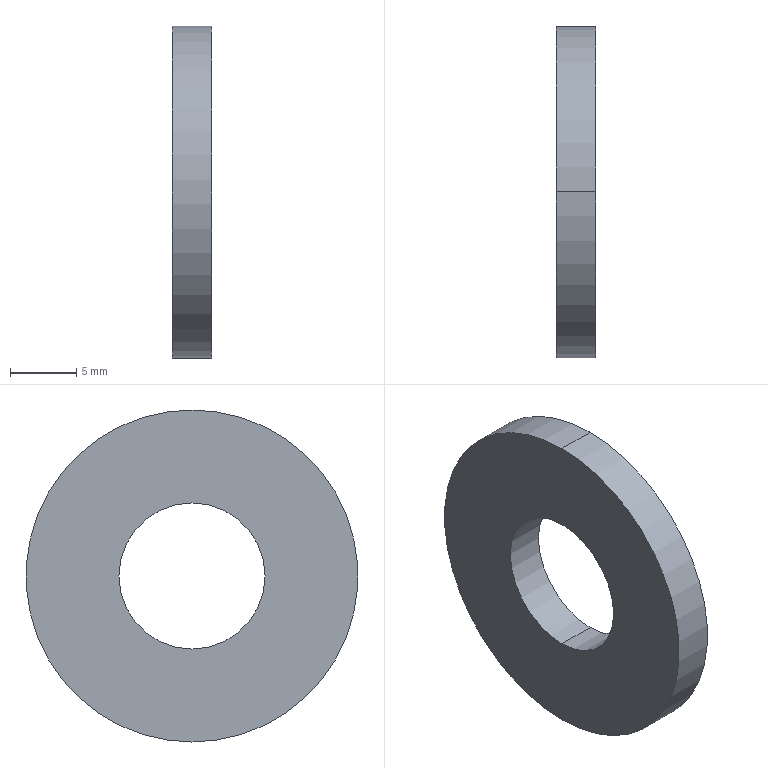Component | SolidWorks | Baffle-1 | 1 solid | 6 faces | box 3 x 25 x 25 mm | volume 1188 mm3 | cylinder 4 | plane 2 | commonest cylinder face diameters 11 x2 25 x2
STEP:
#1=CARTESIAN_POINT('',(7.52,0.7874,3.335));
#2=VERTEX_POINT('',#1);
#3=CARTESIAN_POINT('',(7.52,0.7874,2.902));
#4=VERTEX_POINT('',#3);
#5=CARTESIAN_POINT('',(7.52,0.7874,3.119));
#6=DIRECTION('',(1.,0.,0.));
#7=DIRECTION('',(0.,0.,-1.));
#8=AXIS2_PLACEMENT_3D('',#5,#6,#7);
#9=CIRCLE('',#8,0.2165);
#10=EDGE_CURVE('',#2,#4,#9,.T.);
#11=ORIENTED_EDGE('',*,*,#10,.F.);
#12=CARTESIAN_POINT('',(7.638,0.7874,3.335));
#13=VERTEX_POINT('',#12);
#14=CARTESIAN_POINT('',(7.52,0.7874,3.335));
#15=DIRECTION('',(1.,0.,0.));
#16=VECTOR('',#15,39.37);
#17=LINE('',#14,#16);
#18=EDGE_CURVE('',#2,#13,#17,.T.);
#19=ORIENTED_EDGE('',*,*,#18,.T.);
#20=CARTESIAN_POINT('',(7.638,0.7874,2.902));
#21=VERTEX_POINT('',#20);
#22=CARTESIAN_POINT('',(7.638,0.7874,3.119));
#23=DIRECTION('',(1.,0.,0.));
#24=DIRECTION('',(0.,0.,-1.));
#25=AXIS2_PLACEMENT_3D('',#22,#23,#24);
#26=CIRCLE('',#25,0.2165);
#27=EDGE_CURVE('',#13,#21,#26,.T.);
#28=ORIENTED_EDGE('',*,*,#27,.T.);
#29=CARTESIAN_POINT('',(7.52,0.7874,2.902));
#30=DIRECTION('',(1.,0.,0.));
#31=VECTOR('',#30,39.37);
#32=LINE('',#29,#31);
#33=EDGE_CURVE('',#4,#21,#32,.T.);
#34=ORIENTED_EDGE('',*,*,#33,.F.);
#35=EDGE_LOOP('',(#11,#19,#28,#34));
#36=FACE_OUTER_BOUND('',#35,.T.);
#37=CARTESIAN_POINT('',(7.52,0.7874,3.119));
#38=DIRECTION('',(1.,0.,0.));
#39=DIRECTION('',(0.,0.,-1.));
#40=AXIS2_PLACEMENT_3D('',#37,#38,#39);
#41=CYLINDRICAL_SURFACE('',#40,0.2165);
#42=ADVANCED_FACE('',(#36),#41,.F.);
#43=CARTESIAN_POINT('',(7.52,0.7874,2.626));
#44=VERTEX_POINT('',#43);
#45=CARTESIAN_POINT('',(7.52,0.7874,3.611));
#46=VERTEX_POINT('',#45);
#47=CARTESIAN_POINT('',(7.52,0.7874,3.119));
#48=DIRECTION('',(1.,0.,0.));
#49=DIRECTION('',(0.,0.,-1.));
#50=AXIS2_PLACEMENT_3D('',#47,#48,#49);
#51=CIRCLE('',#50,0.4921);
#52=EDGE_CURVE('',#44,#46,#51,.T.);
#53=ORIENTED_EDGE('',*,*,#52,.T.);
#54=CARTESIAN_POINT('',(7.638,0.7874,3.611));
#55=VERTEX_POINT('',#54);
#56=CARTESIAN_POINT('',(7.52,0.7874,3.611));
#57=DIRECTION('',(1.,0.,0.));
#58=VECTOR('',#57,39.37);
#59=LINE('',#56,#58);
#60=EDGE_CURVE('',#46,#55,#59,.T.);
#61=ORIENTED_EDGE('',*,*,#60,.T.);
#62=CARTESIAN_POINT('',(7.638,0.7874,2.626));
#63=VERTEX_POINT('',#62);
#64=CARTESIAN_POINT('',(7.638,0.7874,3.119));
#65=DIRECTION('',(1.,0.,0.));
#66=DIRECTION('',(0.,0.,-1.));
#67=AXIS2_PLACEMENT_3D('',#64,#65,#66);
#68=CIRCLE('',#67,0.4921);
#69=EDGE_CURVE('',#63,#55,#68,.T.);
#70=ORIENTED_EDGE('',*,*,#69,.F.);
#71=CARTESIAN_POINT('',(7.52,0.7874,2.626));
#72=DIRECTION('',(1.,0.,0.));
#73=VECTOR('',#72,39.37);
#74=LINE('',#71,#73);
#75=EDGE_CURVE('',#44,#63,#74,.T.);
#76=ORIENTED_EDGE('',*,*,#75,.F.);
#77=EDGE_LOOP('',(#53,#61,#70,#76));
#78=FACE_OUTER_BOUND('',#77,.T.);
#79=CARTESIAN_POINT('',(7.52,0.7874,3.119));
#80=DIRECTION('',(1.,0.,0.));
#81=DIRECTION('',(0.,0.,-1.));
#82=AXIS2_PLACEMENT_3D('',#79,#80,#81);
#83=CYLINDRICAL_SURFACE('',#82,0.4921);
#84=ADVANCED_FACE('',(#78),#83,.T.);
#85=ORIENTED_EDGE('',*,*,#60,.F.);
#86=CARTESIAN_POINT('',(7.52,0.7874,3.119));
#87=DIRECTION('',(1.,0.,0.));
#88=DIRECTION('',(0.,0.,-1.));
#89=AXIS2_PLACEMENT_3D('',#86,#87,#88);
#90=CIRCLE('',#89,0.4921);
#91=EDGE_CURVE('',#46,#44,#90,.T.);
#92=ORIENTED_EDGE('',*,*,#91,.T.);
#93=ORIENTED_EDGE('',*,*,#75,.T.);
#94=CARTESIAN_POINT('',(7.638,0.7874,3.119));
#95=DIRECTION('',(1.,0.,0.));
#96=DIRECTION('',(0.,0.,-1.));
#97=AXIS2_PLACEMENT_3D('',#94,#95,#96);
#98=CIRCLE('',#97,0.4921);
#99=EDGE_CURVE('',#55,#63,#98,.T.);
#100=ORIENTED_EDGE('',*,*,#99,.F.);
#101=EDGE_LOOP('',(#85,#92,#93,#100));
#102=FACE_OUTER_BOUND('',#101,.T.);
#103=CARTESIAN_POINT('',(7.52,0.7874,3.119));
#104=DIRECTION('',(1.,0.,0.));
#105=DIRECTION('',(0.,0.,-1.));
#106=AXIS2_PLACEMENT_3D('',#103,#104,#105);
#107=CYLINDRICAL_SURFACE('',#106,0.4921);
#108=ADVANCED_FACE('',(#102),#107,.T.);
#109=CARTESIAN_POINT('',(7.52,0.7874,3.119));
#110=DIRECTION('',(1.,0.,0.));
#111=DIRECTION('',(0.,0.,-1.));
#112=AXIS2_PLACEMENT_3D('',#109,#110,#111);
#113=CIRCLE('',#112,0.2165);
#114=EDGE_CURVE('',#4,#2,#113,.T.);
#115=ORIENTED_EDGE('',*,*,#114,.T.);
#116=ORIENTED_EDGE('',*,*,#10,.T.);
#117=EDGE_LOOP('',(#115,#116));
#118=FACE_BOUND('',#117,.T.);
#119=ORIENTED_EDGE('',*,*,#52,.F.);
#120=ORIENTED_EDGE('',*,*,#91,.F.);
#121=EDGE_LOOP('',(#119,#120));
#122=FACE_OUTER_BOUND('',#121,.T.);
#123=CARTESIAN_POINT('',(7.52,0.7874,3.119));
#124=DIRECTION('',(1.,0.,0.));
#125=DIRECTION('',(0.,0.,-1.));
#126=AXIS2_PLACEMENT_3D('',#123,#124,#125);
#127=PLANE('',#126);
#128=ADVANCED_FACE('',(#118,#122),#127,.F.);
#129=CARTESIAN_POINT('',(7.638,0.7874,3.119));
#130=DIRECTION('',(1.,0.,0.));
#131=DIRECTION('',(0.,0.,-1.));
#132=AXIS2_PLACEMENT_3D('',#129,#130,#131);
#133=CIRCLE('',#132,0.2165);
#134=EDGE_CURVE('',#21,#13,#133,.T.);
#135=ORIENTED_EDGE('',*,*,#134,.F.);
#136=ORIENTED_EDGE('',*,*,#27,.F.);
#137=EDGE_LOOP('',(#135,#136));
#138=FACE_BOUND('',#137,.T.);
#139=ORIENTED_EDGE('',*,*,#69,.T.);
#140=ORIENTED_EDGE('',*,*,#99,.T.);
#141=EDGE_LOOP('',(#139,#140));
#142=FACE_OUTER_BOUND('',#141,.T.);
#143=CARTESIAN_POINT('',(7.638,0.7874,3.119));
#144=DIRECTION('',(1.,0.,0.));
#145=DIRECTION('',(0.,0.,-1.));
#146=AXIS2_PLACEMENT_3D('',#143,#144,#145);
#147=PLANE('',#146);
#148=ADVANCED_FACE('',(#138,#142),#147,.T.);
#149=ORIENTED_EDGE('',*,*,#18,.F.);
#150=ORIENTED_EDGE('',*,*,#114,.F.);
#151=ORIENTED_EDGE('',*,*,#33,.T.);
#152=ORIENTED_EDGE('',*,*,#134,.T.);
#153=EDGE_LOOP('',(#149,#150,#151,#152));
#154=FACE_OUTER_BOUND('',#153,.T.);
#155=CARTESIAN_POINT('',(7.52,0.7874,3.119));
#156=DIRECTION('',(1.,0.,0.));
#157=DIRECTION('',(0.,0.,-1.));
#158=AXIS2_PLACEMENT_3D('',#155,#156,#157);
#159=CYLINDRICAL_SURFACE('',#158,0.2165);
#160=ADVANCED_FACE('',(#154),#159,.F.);
#161=CLOSED_SHELL('',(#42,#84,#108,#128,#148,#160));
#162=MANIFOLD_SOLID_BREP('',#161);
#163=CARTESIAN_POINT('',(0.,0.,0.));
#164=DIRECTION('',(0.,0.,1.));
#165=DIRECTION('',(1.,0.,0.));
#166=AXIS2_PLACEMENT_3D('',#163,#164,#165);
#167=(LENGTH_UNIT()NAMED_UNIT(*)SI_UNIT($,.METRE.));
#168=LENGTH_MEASURE_WITH_UNIT(LENGTH_MEASURE(0.0254),#167);
#169=DIMENSIONAL_EXPONENTS(1.,0.,0.,0.,0.,0.,0.);
#170=(CONVERSION_BASED_UNIT('',#168)LENGTH_UNIT()NAMED_UNIT(#169));
#171=UNCERTAINTY_MEASURE_WITH_UNIT(LENGTH_MEASURE(0.00001),#170,'','');
#172=(NAMED_UNIT(*)PLANE_ANGLE_UNIT()SI_UNIT($,.RADIAN.));
#173=(NAMED_UNIT(*)SI_UNIT($,.STERADIAN.)SOLID_ANGLE_UNIT());
#174=(GEOMETRIC_REPRESENTATION_CONTEXT(3)GLOBAL_UNCERTAINTY_ASSIGNED_CONTEXT((#171))GLOBAL_UNIT_ASSIGNED_CONTEXT((#170,#172,#173))REPRESENTATION_CONTEXT('',''));
#175=ADVANCED_BREP_SHAPE_REPRESENTATION('',(#162,#166),#174);
#176=COLOUR_RGB('',0.7922,0.8196,0.9333);
#177=FILL_AREA_STYLE_COLOUR('',#176);
#178=FILL_AREA_STYLE('',(#177));
#179=SURFACE_STYLE_FILL_AREA(#178);
#180=SURFACE_SIDE_STYLE('',(#179));
#181=SURFACE_STYLE_USAGE(.BOTH.,#180);
#182=PRESENTATION_STYLE_ASSIGNMENT((#181));
#183=STYLED_ITEM('',(#182),#162);
#184=(LENGTH_UNIT()NAMED_UNIT(*)SI_UNIT($,.METRE.));
#185=LENGTH_MEASURE_WITH_UNIT(LENGTH_MEASURE(0.0254),#184);
#186=DIMENSIONAL_EXPONENTS(1.,0.,0.,0.,0.,0.,0.);
#187=(CONVERSION_BASED_UNIT('',#185)LENGTH_UNIT()NAMED_UNIT(#186));
#188=UNCERTAINTY_MEASURE_WITH_UNIT(LENGTH_MEASURE(0.00001),#187,'','');
#189=(NAMED_UNIT(*)PLANE_ANGLE_UNIT()SI_UNIT($,.RADIAN.));
#190=(NAMED_UNIT(*)SI_UNIT($,.STERADIAN.)SOLID_ANGLE_UNIT());
#191=(GEOMETRIC_REPRESENTATION_CONTEXT(3)GLOBAL_UNCERTAINTY_ASSIGNED_CONTEXT((#188))GLOBAL_UNIT_ASSIGNED_CONTEXT((#187,#189,#190))REPRESENTATION_CONTEXT('',''));
#192=MECHANICAL_DESIGN_GEOMETRIC_PRESENTATION_REPRESENTATION('',(#183),#191);
#193=PRESENTATION_LAYER_ASSIGNMENT('','',(#183));